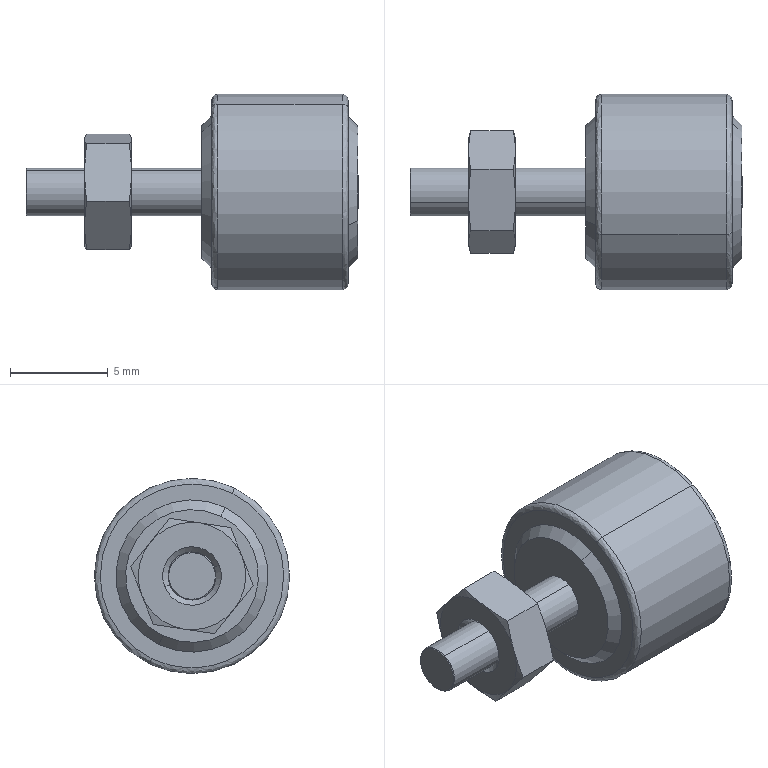Component | SolidWorks | A4-BPF02-3-PP-L-2 | 2 solids | 52 faces | volume 681 mm3 | cone 22 | plane 20 | cylinder 6 | spline 4 | commonest cylinder face diameters 2.459 x4 10 x2